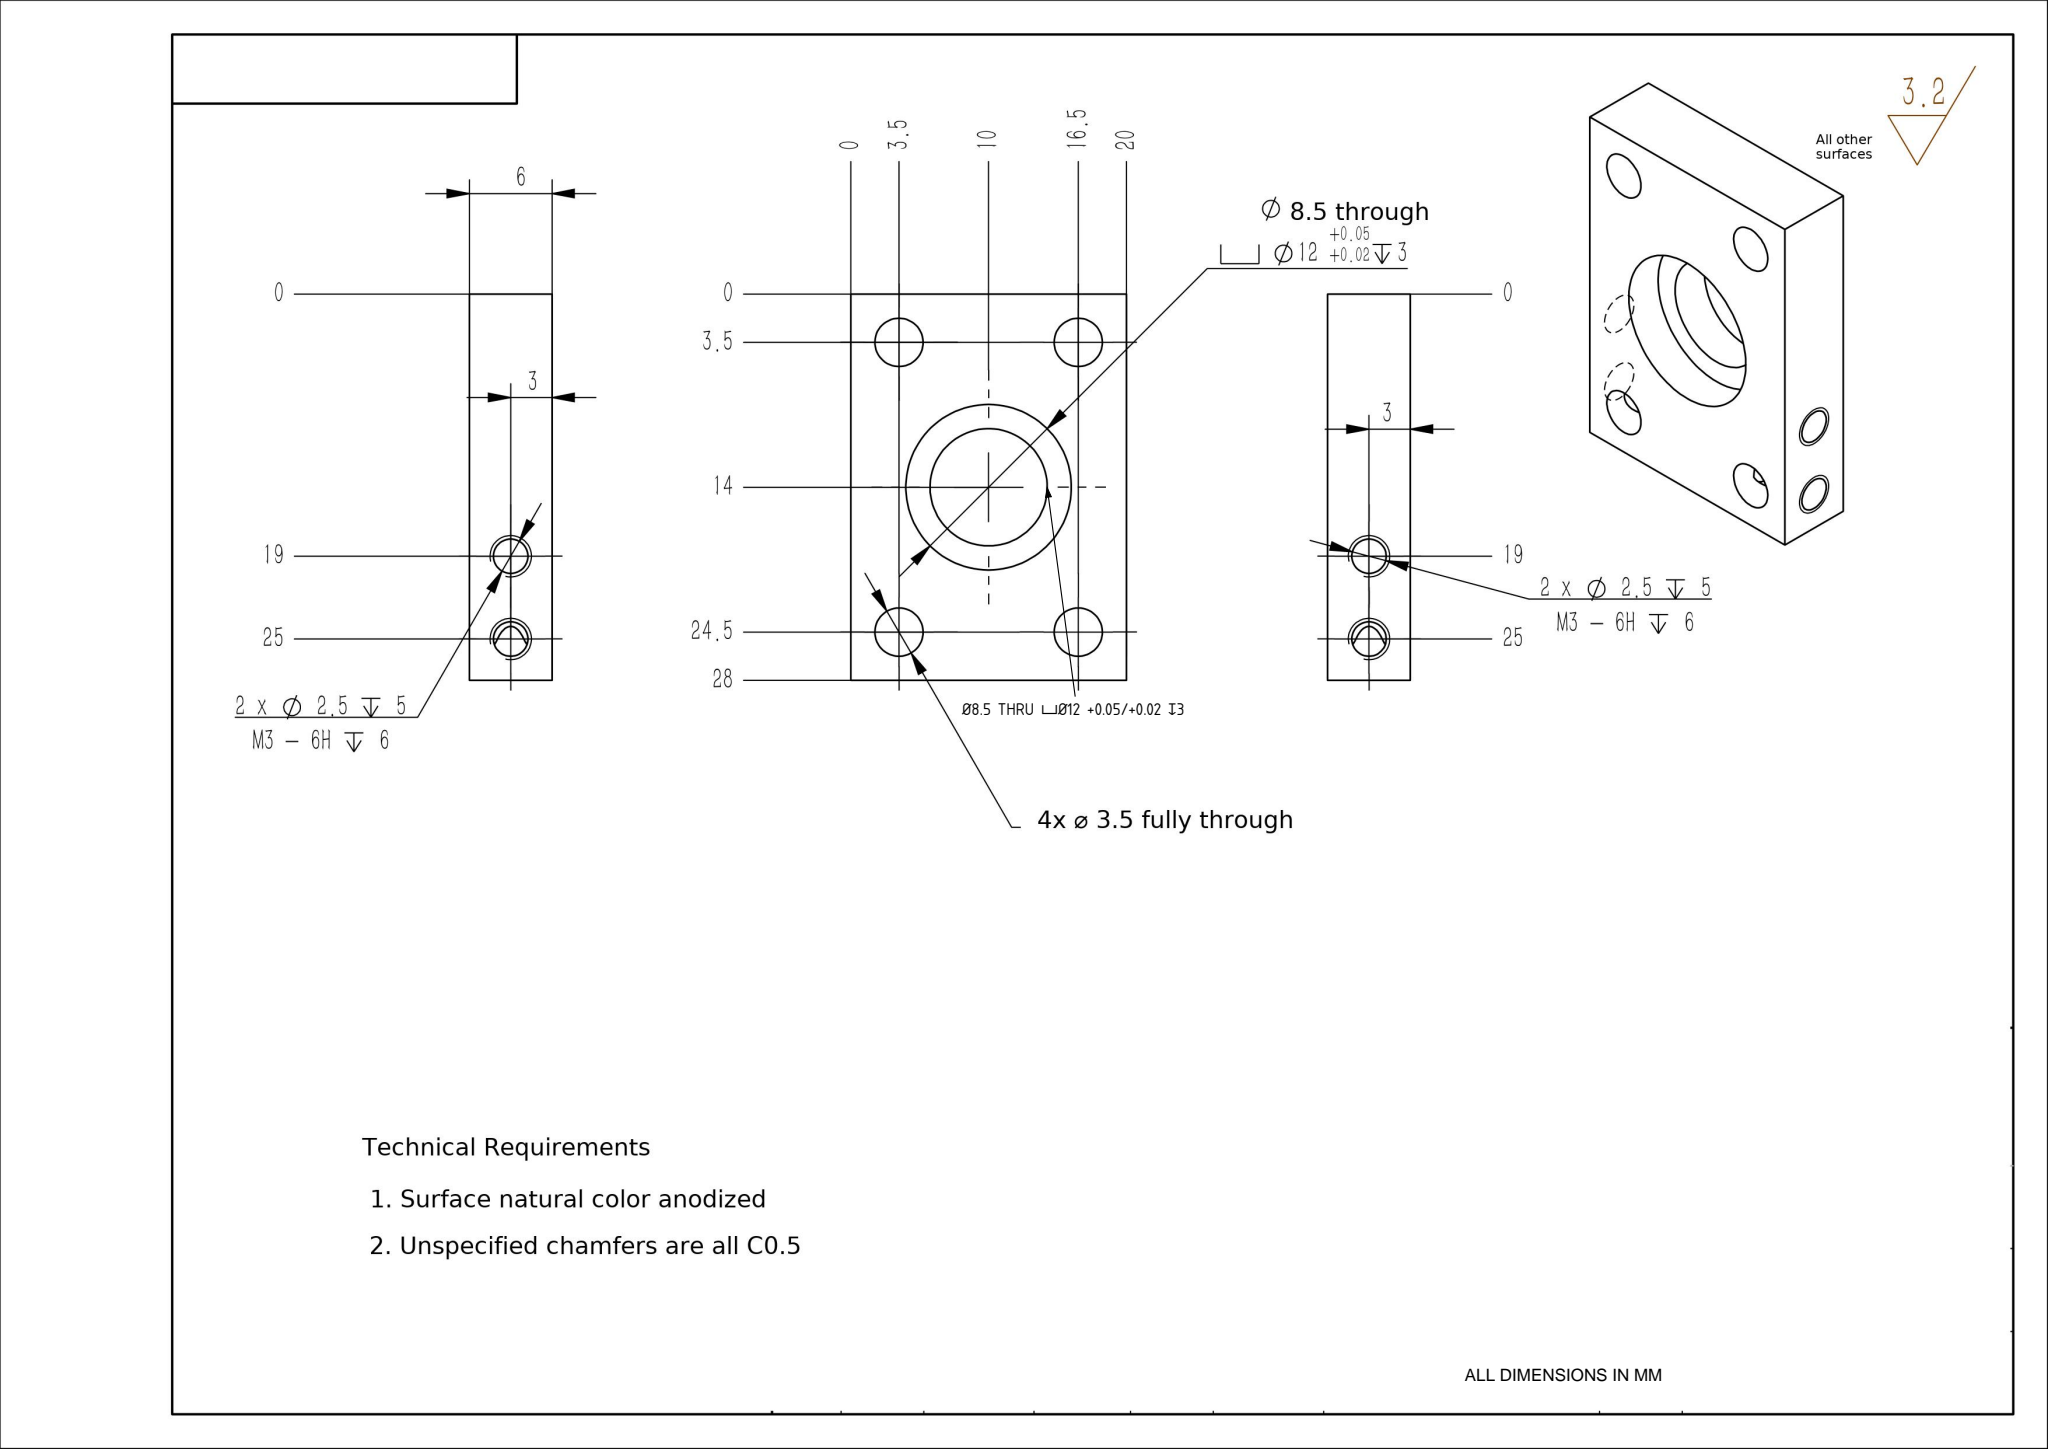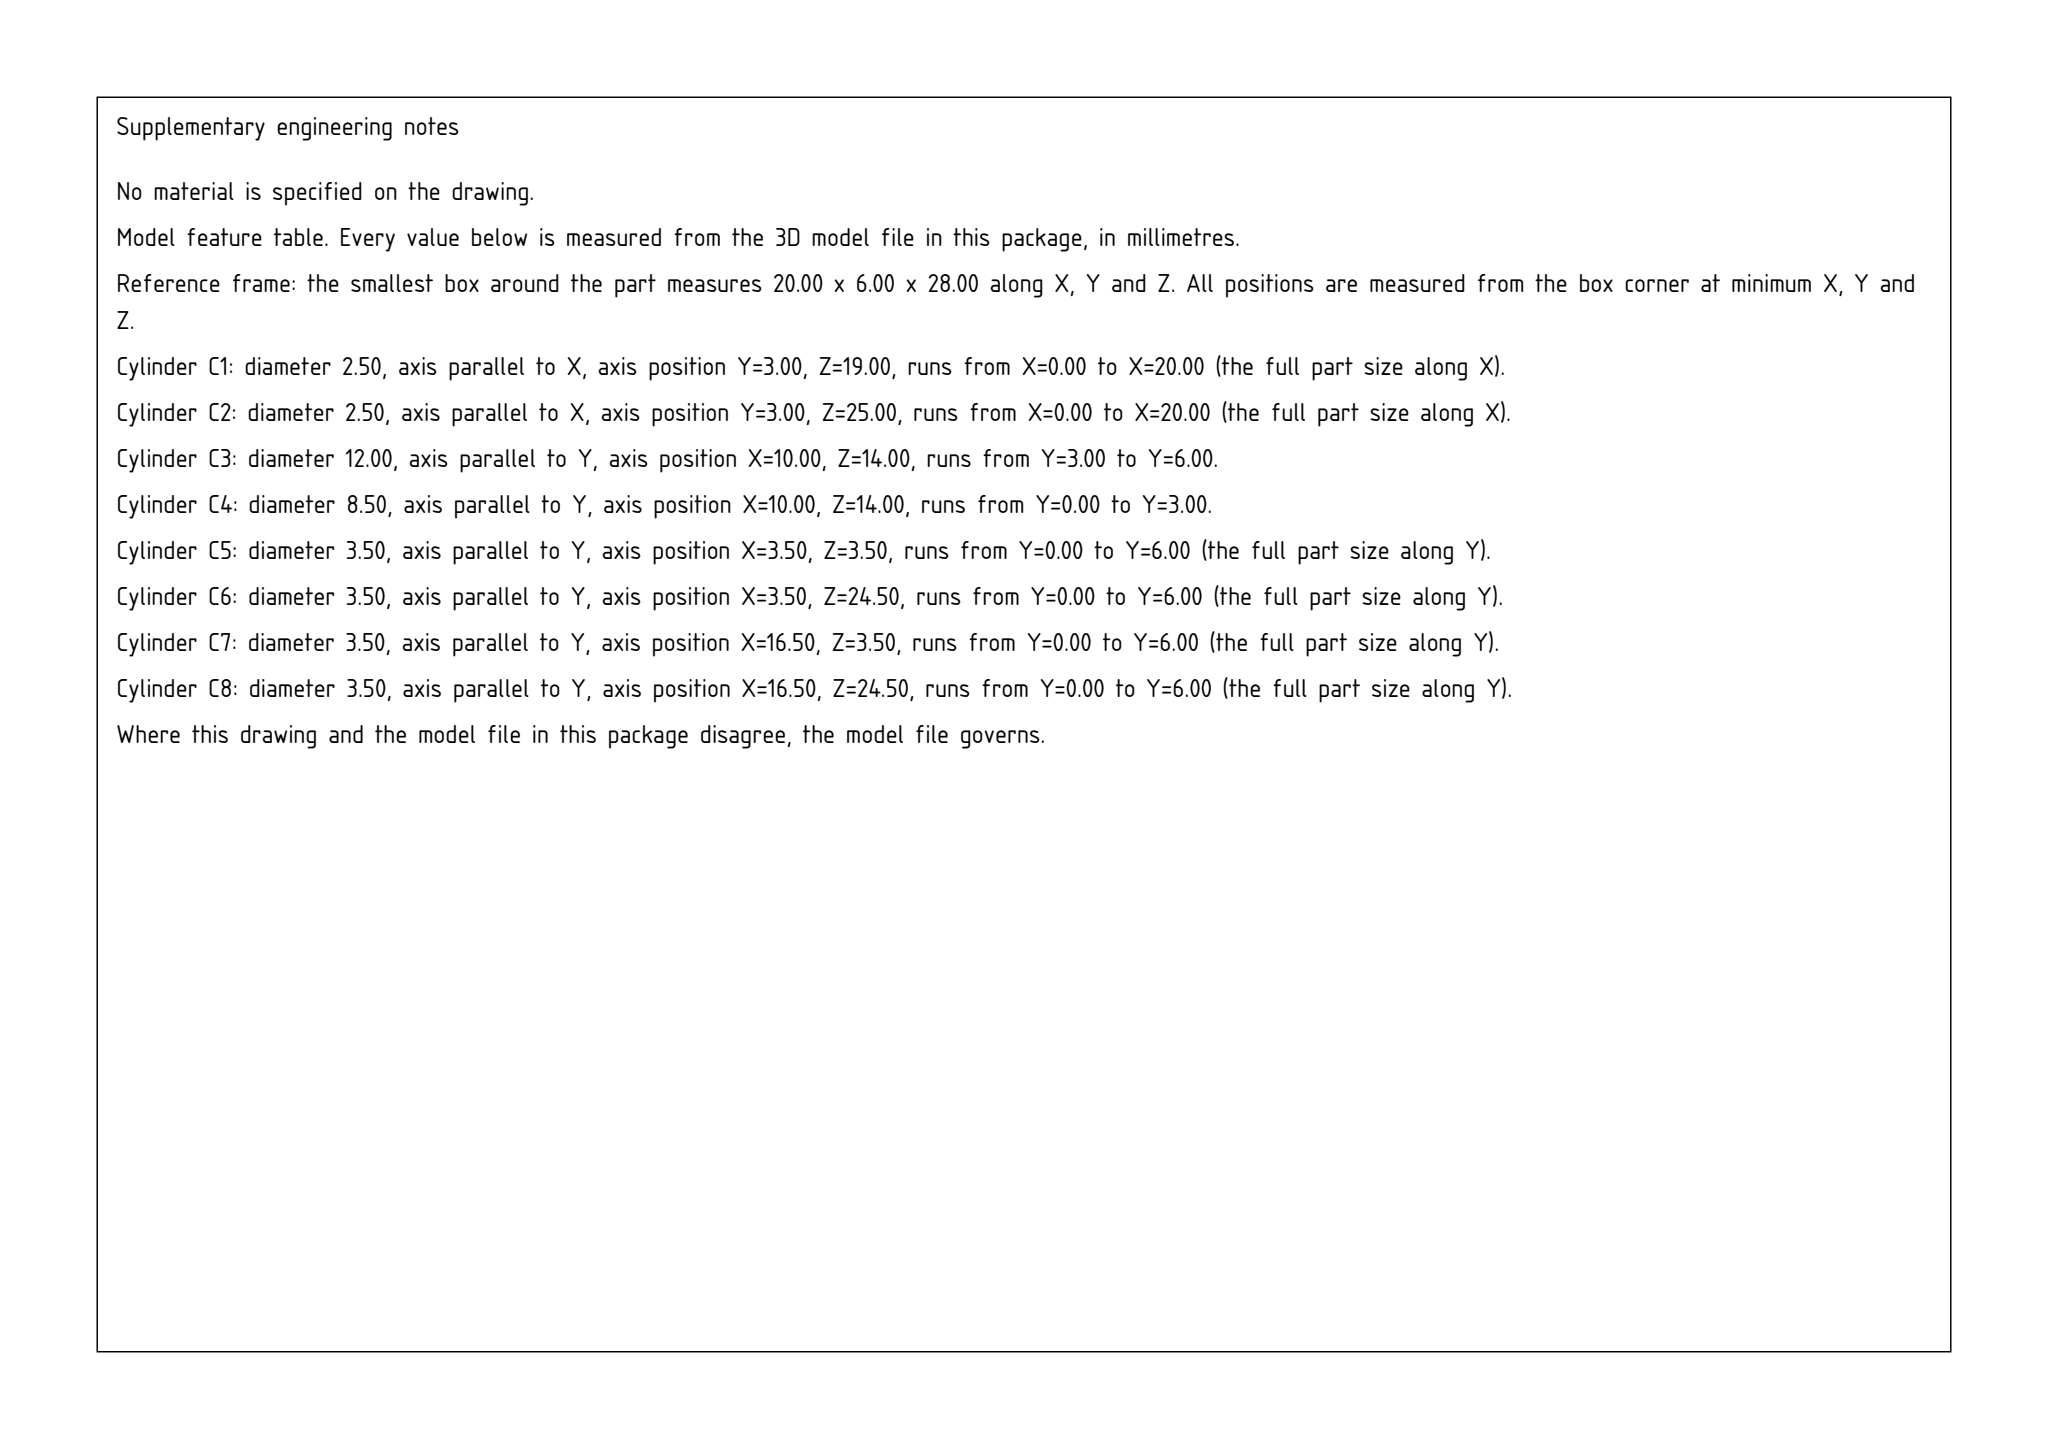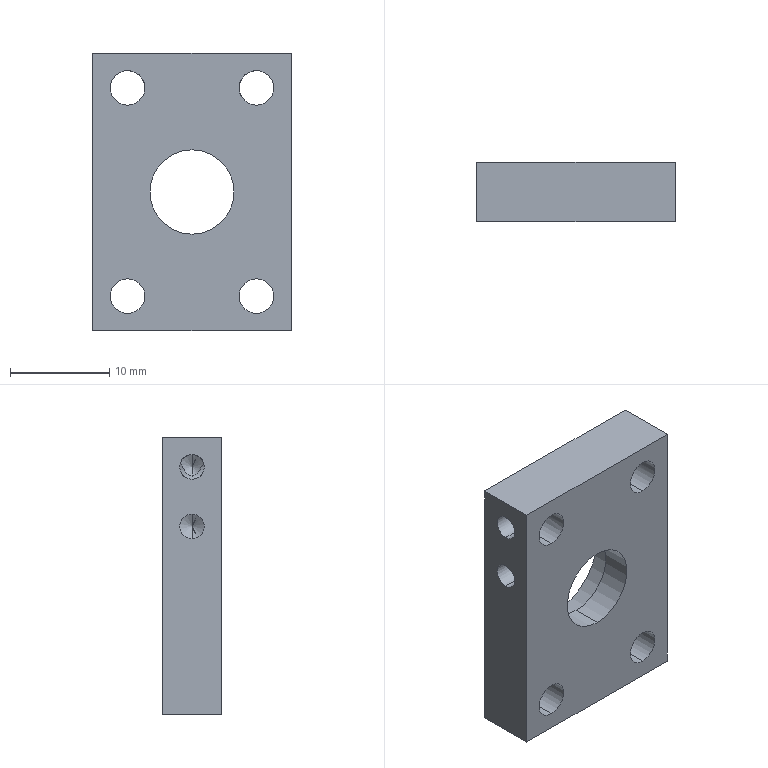Part | SolidWorks | mm | 1 solid | 38 faces | box 20 x 6 x 28 mm | volume 2546 mm3 | cylinder 23 | cone 8 | plane 7 | commonest cylinder face diameters 2.5 x11 3.5 x8 8.5 x2 12 x2
Drawing notes:
Ø8.5 THRU, CBORE Ø12 +0.05/+0.02 DP 3 | from the solid: cyl dia 8.5 axis y len 6 thru at (10,14); cyl dia 12 axis y len 3 at (10,14)
build123d program:
from build123d import *

# Parameters (mm, degrees)
SKETCH1_W                  = 20
SKETCH1_H                  = 28
BOSS_EXTRUDE1_DEPTH        = 6
SKETCH2_R                  = 6
CUT_EXTRUDE1_DEPTH         = 3
SKETCH3_R                  = 4.25
CUT_EXTRUDE2_DEPTH         = 18.464
F_3_5_3_5_DIAMETER_HOLE1_D = 3.5
M3_TAPPED_HOLE1_D          = 2.5
M3_TAPPED_HOLE1_DEPTH      = 5
M3_TAPPED_HOLE1_TIP        = 0.7511
M3_TAPPED_HOLE2_D          = 2.5
M3_TAPPED_HOLE2_DEPTH      = 5
M3_TAPPED_HOLE2_TIP        = 0.7511


with BuildPart() as part:
    # Sketch1 → Boss-Extrude1 (new body)
    with BuildSketch(Plane(origin=(0, 0, 0), x_dir=(1, 0, 0), z_dir=(0, 1, 0))):
        Rectangle(SKETCH1_W, SKETCH1_H)
    extrude(amount=BOSS_EXTRUDE1_DEPTH)

    # Sketch2 → Cut-Extrude1 (cut)
    with BuildSketch(Plane(origin=(0, 6, 0), x_dir=(1, 0, 0), z_dir=(0, 1, 0))):
        with Locations(Location((0, 0, 0), (0, 0, 270))):
            Circle(SKETCH2_R)
    extrude(amount=-CUT_EXTRUDE1_DEPTH, mode=Mode.SUBTRACT)

    # Sketch3 → Cut-Extrude2 (cut, through all)
    with BuildSketch(Plane(origin=(0, 3, 0), x_dir=(1, 0, 0), z_dir=(0, 1, 0))):
        with Locations(Location((0, 0, 0), (0, 0, 270))):
            Circle(SKETCH3_R)
    extrude(amount=-CUT_EXTRUDE2_DEPTH, mode=Mode.SUBTRACT)

    # 3.5 _3.5_ Diameter Hole1 (through all)
    with Locations(Plane(origin=(0, 0, 0), x_dir=(-1, 0, 0), z_dir=(0, -1, 0))):
        with Locations((-6.5, -10.5), (-6.5, 10.5), (6.5, 10.5), (6.5, -10.5)):
            Hole(F_3_5_3_5_DIAMETER_HOLE1_D / 2)

    # M3 Tapped Hole1
    with Locations(Plane.ZY.offset(10)):
        with Locations((11, 3), (5, 3)):
            Hole(M3_TAPPED_HOLE1_D / 2, depth=M3_TAPPED_HOLE1_DEPTH)
            with Locations((0, 0, -(M3_TAPPED_HOLE1_DEPTH + M3_TAPPED_HOLE1_TIP / 2))):  # 118° drill point
                Cone(0, M3_TAPPED_HOLE1_D / 2, M3_TAPPED_HOLE1_TIP, mode=Mode.SUBTRACT)

    # M3 Tapped Hole2
    with Locations(Plane(origin=(10, 0, 0), x_dir=(0, 0, -1), z_dir=(1, 0, 0))):
        with Locations((-5, 3), (-11, 3)):
            Hole(M3_TAPPED_HOLE2_D / 2, depth=M3_TAPPED_HOLE2_DEPTH)
            with Locations((0, 0, -(M3_TAPPED_HOLE2_DEPTH + M3_TAPPED_HOLE2_TIP / 2))):  # 118° drill point
                Cone(0, M3_TAPPED_HOLE2_D / 2, M3_TAPPED_HOLE2_TIP, mode=Mode.SUBTRACT)


solid = part.part